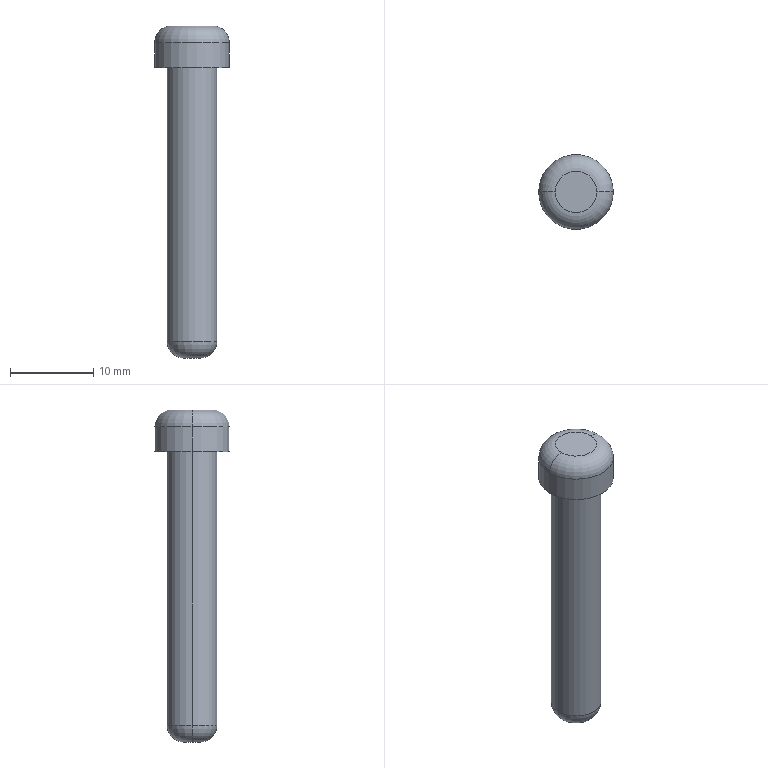Component | SolidWorks | HHL011-1RittalHingePin-2 | 1 solid | 11 faces | box 9 x 9 x 40 mm | volume 1272 mm3 | torus 4 | cylinder 4 | plane 3 | commonest cylinder face diameters 9 x2 6 x2
build123d program:
from build123d import *

# Parameters (mm, degrees)
SKETCH1_R           = 3
BOSS_EXTRUDE1_DEPTH = 35
SKETCH2_R           = 4.5
BOSS_EXTRUDE2_DEPTH = 5
FILLET1_R           = 2
FILLET2_R           = 2


with BuildPart() as part:
    # Sketch1 → Boss-Extrude1 (new body)
    with BuildSketch(Plane.XY):
        with Locations((-18.218, 5.877)):
            Circle(SKETCH1_R)
    extrude(amount=BOSS_EXTRUDE1_DEPTH)

    # Sketch2 → Boss-Extrude2 (add)
    with BuildSketch(Plane.XY.offset(35)):
        with Locations((-18.218, 5.877)):
            Circle(SKETCH2_R)
    extrude(amount=BOSS_EXTRUDE2_DEPTH)

    # Fillet1
    fillet1_edges = [part.edges().sort_by_distance(p)[0] for p in [
        (-22.718, 5.877, 40),
    ]]
    fillet(fillet1_edges, radius=FILLET1_R)

    # Fillet2
    fillet2_edges = [part.edges().sort_by_distance(p)[0] for p in [
        (-21.218, 5.877, 0),
    ]]
    fillet(fillet2_edges, radius=FILLET2_R)


solid = part.part

# Placed as in the assembly
solid = solid.moved(Location((561.194, 169.414, 1432.523), (0, 0, 0)))
STEP:
#1=COLOUR_RGB('',0.7922,0.8196,0.9333);
#2=FILL_AREA_STYLE_COLOUR('',#1);
#3=FILL_AREA_STYLE('',(#2));
#4=SURFACE_STYLE_FILL_AREA(#3);
#5=SURFACE_SIDE_STYLE('',(#4));
#6=SURFACE_STYLE_USAGE(.BOTH.,#5);
#7=PRESENTATION_STYLE_ASSIGNMENT((#6));
#8=CARTESIAN_POINT('',(21.338,6.901,56.399));
#9=VERTEX_POINT('',#8);
#10=CARTESIAN_POINT('',(21.416,6.901,56.399));
#11=VERTEX_POINT('',#10);
#12=CARTESIAN_POINT('',(21.377,6.901,56.399));
#13=DIRECTION('',(0.,0.,-1.));
#14=DIRECTION('',(1.,0.,0.));
#15=AXIS2_PLACEMENT_3D('',#12,#13,#14);
#16=CIRCLE('',#15,0.03937);
#17=EDGE_CURVE('',#9,#11,#16,.T.);
#18=ORIENTED_EDGE('',*,*,#17,.F.);
#19=CARTESIAN_POINT('',(21.259,6.901,56.477));
#20=VERTEX_POINT('',#19);
#21=CARTESIAN_POINT('',(21.338,6.901,56.477));
#22=DIRECTION('',(0.,1.,0.));
#23=DIRECTION('',(-1.,0.,0.));
#24=AXIS2_PLACEMENT_3D('',#21,#22,#23);
#25=CIRCLE('',#24,0.07874);
#26=EDGE_CURVE('',#9,#20,#25,.T.);
#27=ORIENTED_EDGE('',*,*,#26,.T.);
#28=CARTESIAN_POINT('',(21.495,6.901,56.477));
#29=VERTEX_POINT('',#28);
#30=CARTESIAN_POINT('',(21.377,6.901,56.477));
#31=DIRECTION('',(0.,0.,1.));
#32=DIRECTION('',(1.,0.,0.));
#33=AXIS2_PLACEMENT_3D('',#30,#31,#32);
#34=CIRCLE('',#33,0.1181);
#35=EDGE_CURVE('',#29,#20,#34,.T.);
#36=ORIENTED_EDGE('',*,*,#35,.F.);
#37=CARTESIAN_POINT('',(21.416,6.901,56.477));
#38=DIRECTION('',(0.,-1.,0.));
#39=DIRECTION('',(0.,0.,-1.));
#40=AXIS2_PLACEMENT_3D('',#37,#38,#39);
#41=CIRCLE('',#40,0.07874);
#42=EDGE_CURVE('',#11,#29,#41,.T.);
#43=ORIENTED_EDGE('',*,*,#42,.F.);
#44=EDGE_LOOP('',(#18,#27,#36,#43));
#45=FACE_OUTER_BOUND('',#44,.T.);
#46=CARTESIAN_POINT('',(21.377,6.901,56.477));
#47=DIRECTION('',(0.,0.,1.));
#48=DIRECTION('',(1.,0.,0.));
#49=AXIS2_PLACEMENT_3D('',#46,#47,#48);
#50=TOROIDAL_SURFACE('',#49,0.03937,0.07874);
#51=ADVANCED_FACE('',(#45),#50,.T.);
#52=CARTESIAN_POINT('',(21.2,6.901,57.895));
#53=VERTEX_POINT('',#52);
#54=CARTESIAN_POINT('',(21.554,6.901,57.895));
#55=VERTEX_POINT('',#54);
#56=CARTESIAN_POINT('',(21.377,6.901,57.895));
#57=DIRECTION('',(0.,0.,-1.));
#58=DIRECTION('',(1.,0.,0.));
#59=AXIS2_PLACEMENT_3D('',#56,#57,#58);
#60=CIRCLE('',#59,0.1772);
#61=EDGE_CURVE('',#53,#55,#60,.T.);
#62=ORIENTED_EDGE('',*,*,#61,.F.);
#63=CARTESIAN_POINT('',(21.279,6.901,57.973));
#64=VERTEX_POINT('',#63);
#65=CARTESIAN_POINT('',(21.279,6.901,57.895));
#66=DIRECTION('',(0.,1.,0.));
#67=DIRECTION('',(-1.,0.,0.));
#68=AXIS2_PLACEMENT_3D('',#65,#66,#67);
#69=CIRCLE('',#68,0.07874);
#70=EDGE_CURVE('',#53,#64,#69,.T.);
#71=ORIENTED_EDGE('',*,*,#70,.T.);
#72=CARTESIAN_POINT('',(21.475,6.901,57.973));
#73=VERTEX_POINT('',#72);
#74=CARTESIAN_POINT('',(21.377,6.901,57.973));
#75=DIRECTION('',(0.,0.,1.));
#76=DIRECTION('',(1.,0.,0.));
#77=AXIS2_PLACEMENT_3D('',#74,#75,#76);
#78=CIRCLE('',#77,0.09843);
#79=EDGE_CURVE('',#73,#64,#78,.T.);
#80=ORIENTED_EDGE('',*,*,#79,.F.);
#81=CARTESIAN_POINT('',(21.475,6.901,57.895));
#82=DIRECTION('',(0.,-1.,0.));
#83=DIRECTION('',(0.,0.,-1.));
#84=AXIS2_PLACEMENT_3D('',#81,#82,#83);
#85=CIRCLE('',#84,0.07874);
#86=EDGE_CURVE('',#55,#73,#85,.T.);
#87=ORIENTED_EDGE('',*,*,#86,.F.);
#88=EDGE_LOOP('',(#62,#71,#80,#87));
#89=FACE_OUTER_BOUND('',#88,.T.);
#90=CARTESIAN_POINT('',(21.377,6.901,57.895));
#91=DIRECTION('',(0.,0.,1.));
#92=DIRECTION('',(1.,0.,0.));
#93=AXIS2_PLACEMENT_3D('',#90,#91,#92);
#94=TOROIDAL_SURFACE('',#93,0.09843,0.07874);
#95=ADVANCED_FACE('',(#89),#94,.T.);
#96=ORIENTED_EDGE('',*,*,#61,.T.);
#97=CARTESIAN_POINT('',(21.554,6.901,57.777));
#98=VERTEX_POINT('',#97);
#99=CARTESIAN_POINT('',(21.554,6.901,57.973));
#100=DIRECTION('',(0.,0.,-1.));
#101=VECTOR('',#100,39.37);
#102=LINE('',#99,#101);
#103=EDGE_CURVE('',#55,#98,#102,.T.);
#104=ORIENTED_EDGE('',*,*,#103,.T.);
#105=CARTESIAN_POINT('',(21.2,6.901,57.777));
#106=VERTEX_POINT('',#105);
#107=CARTESIAN_POINT('',(21.377,6.901,57.777));
#108=DIRECTION('',(0.,0.,1.));
#109=DIRECTION('',(1.,0.,0.));
#110=AXIS2_PLACEMENT_3D('',#107,#108,#109);
#111=CIRCLE('',#110,0.1772);
#112=EDGE_CURVE('',#98,#106,#111,.T.);
#113=ORIENTED_EDGE('',*,*,#112,.T.);
#114=CARTESIAN_POINT('',(21.2,6.901,57.973));
#115=DIRECTION('',(0.,0.,-1.));
#116=VECTOR('',#115,39.37);
#117=LINE('',#114,#116);
#118=EDGE_CURVE('',#53,#106,#117,.T.);
#119=ORIENTED_EDGE('',*,*,#118,.F.);
#120=EDGE_LOOP('',(#96,#104,#113,#119));
#121=FACE_OUTER_BOUND('',#120,.T.);
#122=CARTESIAN_POINT('',(21.377,6.901,57.973));
#123=DIRECTION('',(0.,0.,-1.));
#124=DIRECTION('',(-1.,0.,0.));
#125=AXIS2_PLACEMENT_3D('',#122,#123,#124);
#126=CYLINDRICAL_SURFACE('',#125,0.1772);
#127=ADVANCED_FACE('',(#121),#126,.T.);
#128=CARTESIAN_POINT('',(21.495,6.901,57.777));
#129=VERTEX_POINT('',#128);
#130=CARTESIAN_POINT('',(21.259,6.901,57.777));
#131=VERTEX_POINT('',#130);
#132=CARTESIAN_POINT('',(21.377,6.901,57.777));
#133=DIRECTION('',(0.,0.,1.));
#134=DIRECTION('',(1.,0.,0.));
#135=AXIS2_PLACEMENT_3D('',#132,#133,#134);
#136=CIRCLE('',#135,0.1181);
#137=EDGE_CURVE('',#129,#131,#136,.T.);
#138=ORIENTED_EDGE('',*,*,#137,.F.);
#139=CARTESIAN_POINT('',(21.495,6.901,57.777));
#140=DIRECTION('',(0.,0.,-1.));
#141=VECTOR('',#140,39.37);
#142=LINE('',#139,#141);
#143=EDGE_CURVE('',#129,#29,#142,.T.);
#144=ORIENTED_EDGE('',*,*,#143,.T.);
#145=ORIENTED_EDGE('',*,*,#35,.T.);
#146=CARTESIAN_POINT('',(21.259,6.901,57.777));
#147=DIRECTION('',(0.,0.,-1.));
#148=VECTOR('',#147,39.37);
#149=LINE('',#146,#148);
#150=EDGE_CURVE('',#131,#20,#149,.T.);
#151=ORIENTED_EDGE('',*,*,#150,.F.);
#152=EDGE_LOOP('',(#138,#144,#145,#151));
#153=FACE_OUTER_BOUND('',#152,.T.);
#154=CARTESIAN_POINT('',(21.377,6.901,57.777));
#155=DIRECTION('',(0.,0.,-1.));
#156=DIRECTION('',(-1.,0.,0.));
#157=AXIS2_PLACEMENT_3D('',#154,#155,#156);
#158=CYLINDRICAL_SURFACE('',#157,0.1181);
#159=ADVANCED_FACE('',(#153),#158,.T.);
#160=ORIENTED_EDGE('',*,*,#143,.F.);
#161=CARTESIAN_POINT('',(21.377,6.901,57.777));
#162=DIRECTION('',(0.,0.,1.));
#163=DIRECTION('',(1.,0.,0.));
#164=AXIS2_PLACEMENT_3D('',#161,#162,#163);
#165=CIRCLE('',#164,0.1181);
#166=EDGE_CURVE('',#131,#129,#165,.T.);
#167=ORIENTED_EDGE('',*,*,#166,.F.);
#168=ORIENTED_EDGE('',*,*,#150,.T.);
#169=CARTESIAN_POINT('',(21.377,6.901,56.477));
#170=DIRECTION('',(0.,0.,1.));
#171=DIRECTION('',(1.,0.,0.));
#172=AXIS2_PLACEMENT_3D('',#169,#170,#171);
#173=CIRCLE('',#172,0.1181);
#174=EDGE_CURVE('',#20,#29,#173,.T.);
#175=ORIENTED_EDGE('',*,*,#174,.T.);
#176=EDGE_LOOP('',(#160,#167,#168,#175));
#177=FACE_OUTER_BOUND('',#176,.T.);
#178=CARTESIAN_POINT('',(21.377,6.901,57.777));
#179=DIRECTION('',(0.,0.,-1.));
#180=DIRECTION('',(-1.,0.,0.));
#181=AXIS2_PLACEMENT_3D('',#178,#179,#180);
#182=CYLINDRICAL_SURFACE('',#181,0.1181);
#183=ADVANCED_FACE('',(#177),#182,.T.);
#184=CARTESIAN_POINT('',(21.377,6.901,56.399));
#185=DIRECTION('',(0.,0.,-1.));
#186=DIRECTION('',(1.,0.,0.));
#187=AXIS2_PLACEMENT_3D('',#184,#185,#186);
#188=CIRCLE('',#187,0.03937);
#189=EDGE_CURVE('',#11,#9,#188,.T.);
#190=ORIENTED_EDGE('',*,*,#189,.T.);
#191=ORIENTED_EDGE('',*,*,#17,.T.);
#192=EDGE_LOOP('',(#190,#191));
#193=FACE_OUTER_BOUND('',#192,.T.);
#194=CARTESIAN_POINT('',(21.377,6.901,56.399));
#195=DIRECTION('',(0.,0.,1.));
#196=DIRECTION('',(1.,0.,0.));
#197=AXIS2_PLACEMENT_3D('',#194,#195,#196);
#198=PLANE('',#197);
#199=ADVANCED_FACE('',(#193),#198,.F.);
#200=CARTESIAN_POINT('',(21.377,6.901,57.777));
#201=DIRECTION('',(0.,0.,1.));
#202=DIRECTION('',(1.,0.,0.));
#203=AXIS2_PLACEMENT_3D('',#200,#201,#202);
#204=CIRCLE('',#203,0.1772);
#205=EDGE_CURVE('',#106,#98,#204,.T.);
#206=ORIENTED_EDGE('',*,*,#205,.F.);
#207=ORIENTED_EDGE('',*,*,#112,.F.);
#208=EDGE_LOOP('',(#206,#207));
#209=FACE_OUTER_BOUND('',#208,.T.);
#210=ORIENTED_EDGE('',*,*,#166,.T.);
#211=ORIENTED_EDGE('',*,*,#137,.T.);
#212=EDGE_LOOP('',(#210,#211));
#213=FACE_BOUND('',#212,.T.);
#214=CARTESIAN_POINT('',(21.377,6.901,57.777));
#215=DIRECTION('',(0.,0.,1.));
#216=DIRECTION('',(1.,0.,0.));
#217=AXIS2_PLACEMENT_3D('',#214,#215,#216);
#218=PLANE('',#217);
#219=ADVANCED_FACE('',(#209,#213),#218,.F.);
#220=ORIENTED_EDGE('',*,*,#103,.F.);
#221=CARTESIAN_POINT('',(21.377,6.901,57.895));
#222=DIRECTION('',(0.,0.,-1.));
#223=DIRECTION('',(1.,0.,0.));
#224=AXIS2_PLACEMENT_3D('',#221,#222,#223);
#225=CIRCLE('',#224,0.1772);
#226=EDGE_CURVE('',#55,#53,#225,.T.);
#227=ORIENTED_EDGE('',*,*,#226,.T.);
#228=ORIENTED_EDGE('',*,*,#118,.T.);
#229=ORIENTED_EDGE('',*,*,#205,.T.);
#230=EDGE_LOOP('',(#220,#227,#228,#229));
#231=FACE_OUTER_BOUND('',#230,.T.);
#232=CARTESIAN_POINT('',(21.377,6.901,57.973));
#233=DIRECTION('',(0.,0.,-1.));
#234=DIRECTION('',(-1.,0.,0.));
#235=AXIS2_PLACEMENT_3D('',#232,#233,#234);
#236=CYLINDRICAL_SURFACE('',#235,0.1772);
#237=ADVANCED_FACE('',(#231),#236,.T.);
#238=ORIENTED_EDGE('',*,*,#79,.T.);
#239=CARTESIAN_POINT('',(21.377,6.901,57.973));
#240=DIRECTION('',(0.,0.,1.));
#241=DIRECTION('',(1.,0.,0.));
#242=AXIS2_PLACEMENT_3D('',#239,#240,#241);
#243=CIRCLE('',#242,0.09843);
#244=EDGE_CURVE('',#64,#73,#243,.T.);
#245=ORIENTED_EDGE('',*,*,#244,.T.);
#246=EDGE_LOOP('',(#238,#245));
#247=FACE_OUTER_BOUND('',#246,.T.);
#248=CARTESIAN_POINT('',(21.377,6.901,57.973));
#249=DIRECTION('',(0.,0.,1.));
#250=DIRECTION('',(1.,0.,0.));
#251=AXIS2_PLACEMENT_3D('',#248,#249,#250);
#252=PLANE('',#251);
#253=ADVANCED_FACE('',(#247),#252,.T.);
#254=ORIENTED_EDGE('',*,*,#70,.F.);
#255=ORIENTED_EDGE('',*,*,#226,.F.);
#256=ORIENTED_EDGE('',*,*,#86,.T.);
#257=ORIENTED_EDGE('',*,*,#244,.F.);
#258=EDGE_LOOP('',(#254,#255,#256,#257));
#259=FACE_OUTER_BOUND('',#258,.T.);
#260=CARTESIAN_POINT('',(21.377,6.901,57.895));
#261=DIRECTION('',(0.,0.,1.));
#262=DIRECTION('',(1.,0.,0.));
#263=AXIS2_PLACEMENT_3D('',#260,#261,#262);
#264=TOROIDAL_SURFACE('',#263,0.09843,0.07874);
#265=ADVANCED_FACE('',(#259),#264,.T.);
#266=ORIENTED_EDGE('',*,*,#26,.F.);
#267=ORIENTED_EDGE('',*,*,#189,.F.);
#268=ORIENTED_EDGE('',*,*,#42,.T.);
#269=ORIENTED_EDGE('',*,*,#174,.F.);
#270=EDGE_LOOP('',(#266,#267,#268,#269));
#271=FACE_OUTER_BOUND('',#270,.T.);
#272=CARTESIAN_POINT('',(21.377,6.901,56.477));
#273=DIRECTION('',(0.,0.,1.));
#274=DIRECTION('',(1.,0.,0.));
#275=AXIS2_PLACEMENT_3D('',#272,#273,#274);
#276=TOROIDAL_SURFACE('',#275,0.03937,0.07874);
#277=ADVANCED_FACE('',(#271),#276,.T.);
#278=CLOSED_SHELL('',(#51,#95,#127,#159,#183,#199,#219,#237,#253,#265,#277));
#279=MANIFOLD_SOLID_BREP('',#278);
#280=STYLED_ITEM('',(#7),#279);
#281=PRESENTATION_LAYER_ASSIGNMENT('','',(#280));
#282=(LENGTH_UNIT()NAMED_UNIT(*)SI_UNIT($,.METRE.));
#283=LENGTH_MEASURE_WITH_UNIT(LENGTH_MEASURE(0.0254),#282);
#284=DIMENSIONAL_EXPONENTS(1.,0.,0.,0.,0.,0.,0.);
#285=(CONVERSION_BASED_UNIT('',#283)LENGTH_UNIT()NAMED_UNIT(#284));
#286=UNCERTAINTY_MEASURE_WITH_UNIT(LENGTH_MEASURE(0.00001),#285,'','');
#287=(NAMED_UNIT(*)PLANE_ANGLE_UNIT()SI_UNIT($,.RADIAN.));
#288=(NAMED_UNIT(*)SI_UNIT($,.STERADIAN.)SOLID_ANGLE_UNIT());
#289=(GEOMETRIC_REPRESENTATION_CONTEXT(3)GLOBAL_UNCERTAINTY_ASSIGNED_CONTEXT((#286))GLOBAL_UNIT_ASSIGNED_CONTEXT((#285,#287,#288))REPRESENTATION_CONTEXT('',''));
#290=MECHANICAL_DESIGN_GEOMETRIC_PRESENTATION_REPRESENTATION('',(#280),#289);
#291=CARTESIAN_POINT('',(0.,0.,0.));
#292=DIRECTION('',(0.,0.,1.));
#293=DIRECTION('',(1.,0.,0.));
#294=AXIS2_PLACEMENT_3D('',#291,#292,#293);
#295=(LENGTH_UNIT()NAMED_UNIT(*)SI_UNIT($,.METRE.));
#296=LENGTH_MEASURE_WITH_UNIT(LENGTH_MEASURE(0.0254),#295);
#297=DIMENSIONAL_EXPONENTS(1.,0.,0.,0.,0.,0.,0.);
#298=(CONVERSION_BASED_UNIT('',#296)LENGTH_UNIT()NAMED_UNIT(#297));
#299=UNCERTAINTY_MEASURE_WITH_UNIT(LENGTH_MEASURE(0.00001),#298,'','');
#300=(NAMED_UNIT(*)PLANE_ANGLE_UNIT()SI_UNIT($,.RADIAN.));
#301=(NAMED_UNIT(*)SI_UNIT($,.STERADIAN.)SOLID_ANGLE_UNIT());
#302=(GEOMETRIC_REPRESENTATION_CONTEXT(3)GLOBAL_UNCERTAINTY_ASSIGNED_CONTEXT((#299))GLOBAL_UNIT_ASSIGNED_CONTEXT((#298,#300,#301))REPRESENTATION_CONTEXT('',''));
#303=ADVANCED_BREP_SHAPE_REPRESENTATION('',(#279,#294),#302);